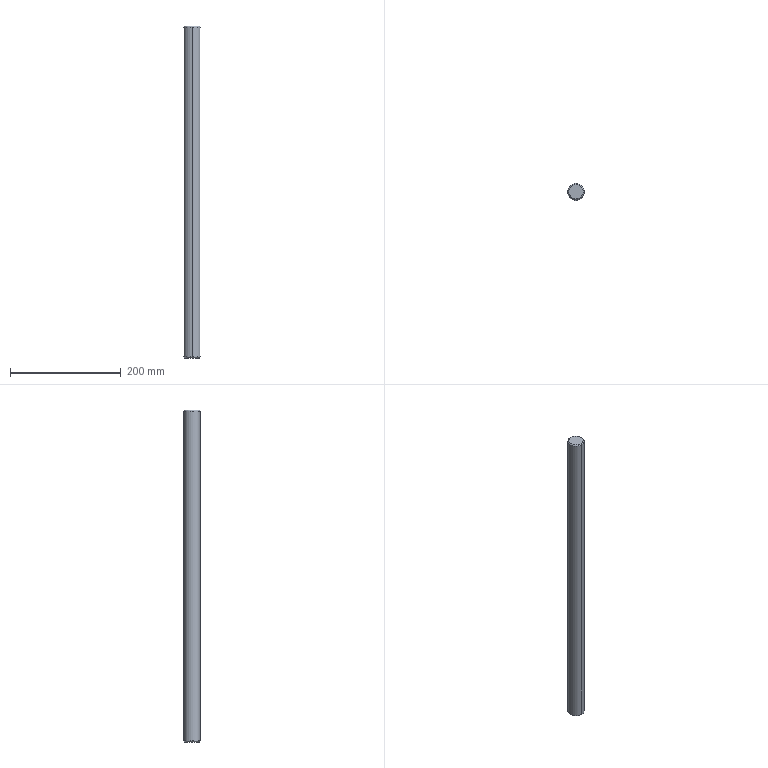Component | SolidWorks | SFTJ-02-Column-1 | 1 solid | 8 faces | box 30 x 30 x 600 mm | volume 423755 mm3 | cone 4 | cylinder 2 | plane 2 | commonest cylinder face diameters 30 x2 | material 45
build123d program:
from build123d import *

# Parameters (mm, degrees)
SKETCH1_R           = 15
BOSS_EXTRUDE1_DEPTH = 300
CHAMFER1_SIZE       = 2


with BuildPart() as part:
    # Sketch1 → Boss-Extrude1 (new, symmetric)
    with BuildSketch(Plane.XY):
        Circle(SKETCH1_R)
    extrude(amount=BOSS_EXTRUDE1_DEPTH, both=True)

    # Chamfer1
    chamfer1_edges = [part.edges().sort_by_distance(p)[0] for p in [
        (-15, 0, -300),
        (-15, 0, 300),
    ]]
    chamfer(chamfer1_edges, length=CHAMFER1_SIZE)


solid = part.part

# Placed as in the assembly
solid = solid.moved(Location((-317.759, -47.279, 253.589), (0, 0, 0)))
STEP:
#1=CARTESIAN_POINT('',(-12.51,-2.373,21.795));
#2=VERTEX_POINT('',#1);
#3=CARTESIAN_POINT('',(-12.51,-1.35,21.795));
#4=VERTEX_POINT('',#3);
#5=CARTESIAN_POINT('',(-12.51,-1.861,21.795));
#6=DIRECTION('',(0.,0.,1.));
#7=DIRECTION('',(0.,-1.,0.));
#8=AXIS2_PLACEMENT_3D('',#5,#6,#7);
#9=CIRCLE('',#8,0.5118);
#10=EDGE_CURVE('',#2,#4,#9,.T.);
#11=ORIENTED_EDGE('',*,*,#10,.F.);
#12=CARTESIAN_POINT('',(-12.51,-2.452,21.716));
#13=VERTEX_POINT('',#12);
#14=CARTESIAN_POINT('',(-12.51,-2.373,21.795));
#15=DIRECTION('',(0.,-0.7071,-0.7071));
#16=VECTOR('',#15,39.37);
#17=LINE('',#14,#16);
#18=EDGE_CURVE('',#2,#13,#17,.T.);
#19=ORIENTED_EDGE('',*,*,#18,.T.);
#20=CARTESIAN_POINT('',(-12.51,-1.271,21.716));
#21=VERTEX_POINT('',#20);
#22=CARTESIAN_POINT('',(-12.51,-1.861,21.716));
#23=DIRECTION('',(0.,0.,-1.));
#24=DIRECTION('',(0.,-1.,0.));
#25=AXIS2_PLACEMENT_3D('',#22,#23,#24);
#26=CIRCLE('',#25,0.5906);
#27=EDGE_CURVE('',#21,#13,#26,.T.);
#28=ORIENTED_EDGE('',*,*,#27,.F.);
#29=CARTESIAN_POINT('',(-12.51,-1.35,21.795));
#30=DIRECTION('',(-0.,0.7071,-0.7071));
#31=VECTOR('',#30,39.37);
#32=LINE('',#29,#31);
#33=EDGE_CURVE('',#4,#21,#32,.T.);
#34=ORIENTED_EDGE('',*,*,#33,.F.);
#35=EDGE_LOOP('',(#11,#19,#28,#34));
#36=FACE_OUTER_BOUND('',#35,.T.);
#37=CARTESIAN_POINT('',(-12.51,-1.861,21.795));
#38=DIRECTION('',(0.,0.,-1.));
#39=DIRECTION('',(0.,1.,0.));
#40=AXIS2_PLACEMENT_3D('',#37,#38,#39);
#41=CONICAL_SURFACE('',#40,0.5118,0.7854);
#42=ADVANCED_FACE('',(#36),#41,.T.);
#43=CARTESIAN_POINT('',(-12.51,-1.35,-1.827));
#44=VERTEX_POINT('',#43);
#45=CARTESIAN_POINT('',(-12.51,-2.373,-1.827));
#46=VERTEX_POINT('',#45);
#47=CARTESIAN_POINT('',(-12.51,-1.861,-1.827));
#48=DIRECTION('',(0.,0.,-1.));
#49=DIRECTION('',(0.,-1.,0.));
#50=AXIS2_PLACEMENT_3D('',#47,#48,#49);
#51=CIRCLE('',#50,0.5118);
#52=EDGE_CURVE('',#44,#46,#51,.T.);
#53=ORIENTED_EDGE('',*,*,#52,.F.);
#54=CARTESIAN_POINT('',(-12.51,-1.271,-1.748));
#55=VERTEX_POINT('',#54);
#56=CARTESIAN_POINT('',(-12.51,-1.271,-1.748));
#57=DIRECTION('',(0.,0.7071,0.7071));
#58=VECTOR('',#57,39.37);
#59=LINE('',#56,#58);
#60=EDGE_CURVE('',#44,#55,#59,.T.);
#61=ORIENTED_EDGE('',*,*,#60,.T.);
#62=CARTESIAN_POINT('',(-12.51,-2.452,-1.748));
#63=VERTEX_POINT('',#62);
#64=CARTESIAN_POINT('',(-12.51,-1.861,-1.748));
#65=DIRECTION('',(0.,0.,1.));
#66=DIRECTION('',(0.,-1.,0.));
#67=AXIS2_PLACEMENT_3D('',#64,#65,#66);
#68=CIRCLE('',#67,0.5906);
#69=EDGE_CURVE('',#63,#55,#68,.T.);
#70=ORIENTED_EDGE('',*,*,#69,.F.);
#71=CARTESIAN_POINT('',(-12.51,-2.452,-1.748));
#72=DIRECTION('',(0.,-0.7071,0.7071));
#73=VECTOR('',#72,39.37);
#74=LINE('',#71,#73);
#75=EDGE_CURVE('',#46,#63,#74,.T.);
#76=ORIENTED_EDGE('',*,*,#75,.F.);
#77=EDGE_LOOP('',(#53,#61,#70,#76));
#78=FACE_OUTER_BOUND('',#77,.T.);
#79=CARTESIAN_POINT('',(-12.51,-1.861,-1.748));
#80=DIRECTION('',(0.,0.,1.));
#81=DIRECTION('',(0.,-1.,0.));
#82=AXIS2_PLACEMENT_3D('',#79,#80,#81);
#83=CONICAL_SURFACE('',#82,0.5906,0.7854);
#84=ADVANCED_FACE('',(#78),#83,.T.);
#85=ORIENTED_EDGE('',*,*,#27,.T.);
#86=CARTESIAN_POINT('',(-12.51,-2.452,21.795));
#87=DIRECTION('',(0.,0.,-1.));
#88=VECTOR('',#87,39.37);
#89=LINE('',#86,#88);
#90=EDGE_CURVE('',#13,#63,#89,.T.);
#91=ORIENTED_EDGE('',*,*,#90,.T.);
#92=ORIENTED_EDGE('',*,*,#69,.T.);
#93=CARTESIAN_POINT('',(-12.51,-1.271,21.795));
#94=DIRECTION('',(0.,0.,-1.));
#95=VECTOR('',#94,39.37);
#96=LINE('',#93,#95);
#97=EDGE_CURVE('',#21,#55,#96,.T.);
#98=ORIENTED_EDGE('',*,*,#97,.F.);
#99=EDGE_LOOP('',(#85,#91,#92,#98));
#100=FACE_OUTER_BOUND('',#99,.T.);
#101=CARTESIAN_POINT('',(-12.51,-1.861,21.795));
#102=DIRECTION('',(0.,0.,-1.));
#103=DIRECTION('',(0.,1.,0.));
#104=AXIS2_PLACEMENT_3D('',#101,#102,#103);
#105=CYLINDRICAL_SURFACE('',#104,0.5906);
#106=ADVANCED_FACE('',(#100),#105,.T.);
#107=ORIENTED_EDGE('',*,*,#90,.F.);
#108=CARTESIAN_POINT('',(-12.51,-1.861,21.716));
#109=DIRECTION('',(0.,0.,-1.));
#110=DIRECTION('',(0.,-1.,0.));
#111=AXIS2_PLACEMENT_3D('',#108,#109,#110);
#112=CIRCLE('',#111,0.5906);
#113=EDGE_CURVE('',#13,#21,#112,.T.);
#114=ORIENTED_EDGE('',*,*,#113,.T.);
#115=ORIENTED_EDGE('',*,*,#97,.T.);
#116=CARTESIAN_POINT('',(-12.51,-1.861,-1.748));
#117=DIRECTION('',(0.,0.,1.));
#118=DIRECTION('',(0.,-1.,0.));
#119=AXIS2_PLACEMENT_3D('',#116,#117,#118);
#120=CIRCLE('',#119,0.5906);
#121=EDGE_CURVE('',#55,#63,#120,.T.);
#122=ORIENTED_EDGE('',*,*,#121,.T.);
#123=EDGE_LOOP('',(#107,#114,#115,#122));
#124=FACE_OUTER_BOUND('',#123,.T.);
#125=CARTESIAN_POINT('',(-12.51,-1.861,21.795));
#126=DIRECTION('',(0.,0.,-1.));
#127=DIRECTION('',(0.,1.,0.));
#128=AXIS2_PLACEMENT_3D('',#125,#126,#127);
#129=CYLINDRICAL_SURFACE('',#128,0.5906);
#130=ADVANCED_FACE('',(#124),#129,.T.);
#131=CARTESIAN_POINT('',(-12.51,-1.861,21.795));
#132=DIRECTION('',(0.,0.,1.));
#133=DIRECTION('',(0.,-1.,0.));
#134=AXIS2_PLACEMENT_3D('',#131,#132,#133);
#135=CIRCLE('',#134,0.5118);
#136=EDGE_CURVE('',#4,#2,#135,.T.);
#137=ORIENTED_EDGE('',*,*,#136,.T.);
#138=ORIENTED_EDGE('',*,*,#10,.T.);
#139=EDGE_LOOP('',(#137,#138));
#140=FACE_OUTER_BOUND('',#139,.T.);
#141=CARTESIAN_POINT('',(-12.51,-1.861,21.795));
#142=DIRECTION('',(0.,0.,1.));
#143=DIRECTION('',(0.,-1.,0.));
#144=AXIS2_PLACEMENT_3D('',#141,#142,#143);
#145=PLANE('',#144);
#146=ADVANCED_FACE('',(#140),#145,.T.);
#147=CARTESIAN_POINT('',(-12.51,-1.861,-1.827));
#148=DIRECTION('',(0.,0.,-1.));
#149=DIRECTION('',(0.,-1.,0.));
#150=AXIS2_PLACEMENT_3D('',#147,#148,#149);
#151=CIRCLE('',#150,0.5118);
#152=EDGE_CURVE('',#46,#44,#151,.T.);
#153=ORIENTED_EDGE('',*,*,#152,.T.);
#154=ORIENTED_EDGE('',*,*,#52,.T.);
#155=EDGE_LOOP('',(#153,#154));
#156=FACE_OUTER_BOUND('',#155,.T.);
#157=CARTESIAN_POINT('',(-12.51,-1.861,-1.827));
#158=DIRECTION('',(0.,0.,1.));
#159=DIRECTION('',(0.,-1.,0.));
#160=AXIS2_PLACEMENT_3D('',#157,#158,#159);
#161=PLANE('',#160);
#162=ADVANCED_FACE('',(#156),#161,.F.);
#163=ORIENTED_EDGE('',*,*,#60,.F.);
#164=ORIENTED_EDGE('',*,*,#152,.F.);
#165=ORIENTED_EDGE('',*,*,#75,.T.);
#166=ORIENTED_EDGE('',*,*,#121,.F.);
#167=EDGE_LOOP('',(#163,#164,#165,#166));
#168=FACE_OUTER_BOUND('',#167,.T.);
#169=CARTESIAN_POINT('',(-12.51,-1.861,-1.748));
#170=DIRECTION('',(0.,0.,1.));
#171=DIRECTION('',(0.,-1.,0.));
#172=AXIS2_PLACEMENT_3D('',#169,#170,#171);
#173=CONICAL_SURFACE('',#172,0.5906,0.7854);
#174=ADVANCED_FACE('',(#168),#173,.T.);
#175=ORIENTED_EDGE('',*,*,#18,.F.);
#176=ORIENTED_EDGE('',*,*,#136,.F.);
#177=ORIENTED_EDGE('',*,*,#33,.T.);
#178=ORIENTED_EDGE('',*,*,#113,.F.);
#179=EDGE_LOOP('',(#175,#176,#177,#178));
#180=FACE_OUTER_BOUND('',#179,.T.);
#181=CARTESIAN_POINT('',(-12.51,-1.861,21.795));
#182=DIRECTION('',(0.,0.,-1.));
#183=DIRECTION('',(0.,1.,0.));
#184=AXIS2_PLACEMENT_3D('',#181,#182,#183);
#185=CONICAL_SURFACE('',#184,0.5118,0.7854);
#186=ADVANCED_FACE('',(#180),#185,.T.);
#187=CLOSED_SHELL('',(#42,#84,#106,#130,#146,#162,#174,#186));
#188=MANIFOLD_SOLID_BREP('',#187);
#189=CARTESIAN_POINT('',(0.,0.,0.));
#190=DIRECTION('',(0.,0.,1.));
#191=DIRECTION('',(1.,0.,0.));
#192=AXIS2_PLACEMENT_3D('',#189,#190,#191);
#193=(LENGTH_UNIT()NAMED_UNIT(*)SI_UNIT($,.METRE.));
#194=LENGTH_MEASURE_WITH_UNIT(LENGTH_MEASURE(0.0254),#193);
#195=DIMENSIONAL_EXPONENTS(1.,0.,0.,0.,0.,0.,0.);
#196=(CONVERSION_BASED_UNIT('',#194)LENGTH_UNIT()NAMED_UNIT(#195));
#197=UNCERTAINTY_MEASURE_WITH_UNIT(LENGTH_MEASURE(0.00001),#196,'','');
#198=(NAMED_UNIT(*)PLANE_ANGLE_UNIT()SI_UNIT($,.RADIAN.));
#199=(NAMED_UNIT(*)SI_UNIT($,.STERADIAN.)SOLID_ANGLE_UNIT());
#200=(GEOMETRIC_REPRESENTATION_CONTEXT(3)GLOBAL_UNCERTAINTY_ASSIGNED_CONTEXT((#197))GLOBAL_UNIT_ASSIGNED_CONTEXT((#196,#198,#199))REPRESENTATION_CONTEXT('',''));
#201=ADVANCED_BREP_SHAPE_REPRESENTATION('',(#188,#192),#200);
#202=COLOUR_RGB('',0.7922,0.8196,0.9333);
#203=FILL_AREA_STYLE_COLOUR('',#202);
#204=FILL_AREA_STYLE('',(#203));
#205=SURFACE_STYLE_FILL_AREA(#204);
#206=SURFACE_SIDE_STYLE('',(#205));
#207=SURFACE_STYLE_USAGE(.BOTH.,#206);
#208=PRESENTATION_STYLE_ASSIGNMENT((#207));
#209=STYLED_ITEM('',(#208),#188);
#210=(LENGTH_UNIT()NAMED_UNIT(*)SI_UNIT($,.METRE.));
#211=LENGTH_MEASURE_WITH_UNIT(LENGTH_MEASURE(0.0254),#210);
#212=DIMENSIONAL_EXPONENTS(1.,0.,0.,0.,0.,0.,0.);
#213=(CONVERSION_BASED_UNIT('',#211)LENGTH_UNIT()NAMED_UNIT(#212));
#214=UNCERTAINTY_MEASURE_WITH_UNIT(LENGTH_MEASURE(0.00001),#213,'','');
#215=(NAMED_UNIT(*)PLANE_ANGLE_UNIT()SI_UNIT($,.RADIAN.));
#216=(NAMED_UNIT(*)SI_UNIT($,.STERADIAN.)SOLID_ANGLE_UNIT());
#217=(GEOMETRIC_REPRESENTATION_CONTEXT(3)GLOBAL_UNCERTAINTY_ASSIGNED_CONTEXT((#214))GLOBAL_UNIT_ASSIGNED_CONTEXT((#213,#215,#216))REPRESENTATION_CONTEXT('',''));
#218=MECHANICAL_DESIGN_GEOMETRIC_PRESENTATION_REPRESENTATION('',(#209),#217);
#219=PRESENTATION_LAYER_ASSIGNMENT('','',(#209));